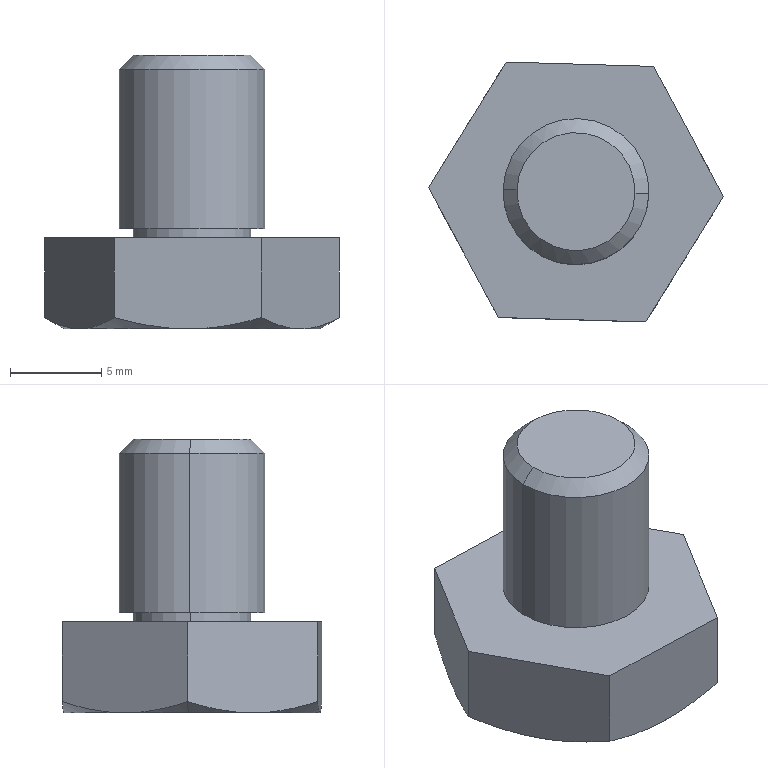Component | SolidWorks | STEHN14-1 | 1 solid | 23 faces | box 16.16 x 14.23 x 15 mm | volume 1333 mm3 | plane 10 | cone 9 | cylinder 4 | commonest cylinder face diameters 8 x2 6.466 x2 | material SUJ2
STEP:
#1=COLOUR_RGB('',0.7922,0.8196,0.9333);
#2=FILL_AREA_STYLE_COLOUR('',#1);
#3=FILL_AREA_STYLE('',(#2));
#4=SURFACE_STYLE_FILL_AREA(#3);
#5=SURFACE_SIDE_STYLE('',(#4));
#6=SURFACE_STYLE_USAGE(.BOTH.,#5);
#7=PRESENTATION_STYLE_ASSIGNMENT((#6));
#8=CARTESIAN_POINT('',(17.281,6.304,-9.769));
#9=VERTEX_POINT('',#8);
#10=CARTESIAN_POINT('',(17.322,6.441,-9.769));
#11=VERTEX_POINT('',#10);
#12=CARTESIAN_POINT('',(17.556,6.296,-9.769));
#13=DIRECTION('',(0.,-0.,-1.));
#14=DIRECTION('',(0.9996,-0.02982,0.));
#15=AXIS2_PLACEMENT_3D('',#12,#13,#14);
#16=CIRCLE('',#15,0.2756);
#17=EDGE_CURVE('',#9,#11,#16,.T.);
#18=ORIENTED_EDGE('',*,*,#17,.F.);
#19=CARTESIAN_POINT('',(17.238,6.305,-9.744));
#20=VERTEX_POINT('',#19);
#21=CARTESIAN_POINT('',(17.237,6.305,-9.744));
#22=DIRECTION('',(-0.8656,0.02582,0.5));
#23=VECTOR('',#22,39.37);
#24=LINE('',#21,#23);
#25=EDGE_CURVE('',#9,#20,#24,.T.);
#26=ORIENTED_EDGE('',*,*,#25,.T.);
#27=CARTESIAN_POINT('',(17.322,6.441,-9.769));
#28=CARTESIAN_POINT('',(17.315,6.429,-9.769));
#29=CARTESIAN_POINT('',(17.307,6.418,-9.768));
#30=CARTESIAN_POINT('',(17.293,6.395,-9.766));
#31=CARTESIAN_POINT('',(17.286,6.384,-9.764));
#32=CARTESIAN_POINT('',(17.265,6.35,-9.758));
#33=CARTESIAN_POINT('',(17.252,6.327,-9.752));
#34=CARTESIAN_POINT('',(17.238,6.305,-9.744));
#35=B_SPLINE_CURVE_WITH_KNOTS('',3,(#27,#28,#29,#30,#31,#32,#33,#34),.UNSPECIFIED.,.F.,.F.,(4,2,2,4),(0.00409,0.005108,0.006127,0.008164),.UNSPECIFIED.);
#36=EDGE_CURVE('',#11,#20,#35,.T.);
#37=ORIENTED_EDGE('',*,*,#36,.F.);
#38=EDGE_LOOP('',(#18,#26,#37));
#39=FACE_OUTER_BOUND('',#38,.T.);
#40=CARTESIAN_POINT('',(17.556,6.296,-9.744));
#41=DIRECTION('',(-0.,0.,1.));
#42=DIRECTION('',(-0.9996,0.02982,0.));
#43=AXIS2_PLACEMENT_3D('',#40,#41,#42);
#44=CONICAL_SURFACE('',#43,0.3189,1.047);
#45=ADVANCED_FACE('',(#39),#44,.T.);
#46=CARTESIAN_POINT('',(17.683,6.292,-9.178));
#47=VERTEX_POINT('',#46);
#48=CARTESIAN_POINT('',(17.429,6.3,-9.178));
#49=VERTEX_POINT('',#48);
#50=CARTESIAN_POINT('',(17.556,6.296,-9.178));
#51=DIRECTION('',(0.,-0.,-1.));
#52=DIRECTION('',(0.9996,-0.02982,0.));
#53=AXIS2_PLACEMENT_3D('',#50,#51,#52);
#54=CIRCLE('',#53,0.1273);
#55=EDGE_CURVE('',#47,#49,#54,.T.);
#56=ORIENTED_EDGE('',*,*,#55,.T.);
#57=CARTESIAN_POINT('',(17.399,6.301,-9.209));
#58=VERTEX_POINT('',#57);
#59=CARTESIAN_POINT('',(17.429,6.3,-9.178));
#60=DIRECTION('',(-0.7068,0.02108,-0.7071));
#61=VECTOR('',#60,39.37);
#62=LINE('',#59,#61);
#63=EDGE_CURVE('',#49,#58,#62,.T.);
#64=ORIENTED_EDGE('',*,*,#63,.T.);
#65=CARTESIAN_POINT('',(17.714,6.291,-9.209));
#66=VERTEX_POINT('',#65);
#67=CARTESIAN_POINT('',(17.556,6.296,-9.209));
#68=DIRECTION('',(0.,-0.,-1.));
#69=DIRECTION('',(0.9996,-0.02982,0.));
#70=AXIS2_PLACEMENT_3D('',#67,#68,#69);
#71=CIRCLE('',#70,0.1575);
#72=EDGE_CURVE('',#66,#58,#71,.T.);
#73=ORIENTED_EDGE('',*,*,#72,.F.);
#74=CARTESIAN_POINT('',(17.683,6.292,-9.178));
#75=DIRECTION('',(0.7068,-0.02108,-0.7071));
#76=VECTOR('',#75,39.37);
#77=LINE('',#74,#76);
#78=EDGE_CURVE('',#47,#66,#77,.T.);
#79=ORIENTED_EDGE('',*,*,#78,.F.);
#80=EDGE_LOOP('',(#56,#64,#73,#79));
#81=FACE_OUTER_BOUND('',#80,.T.);
#82=CARTESIAN_POINT('',(17.556,6.296,-9.178));
#83=DIRECTION('',(0.,-0.,-1.));
#84=DIRECTION('',(0.9996,-0.02982,0.));
#85=AXIS2_PLACEMENT_3D('',#82,#83,#84);
#86=CONICAL_SURFACE('',#85,0.1273,0.7854);
#87=ADVANCED_FACE('',(#81),#86,.T.);
#88=ORIENTED_EDGE('',*,*,#72,.T.);
#89=CARTESIAN_POINT('',(17.399,6.301,-9.552));
#90=VERTEX_POINT('',#89);
#91=CARTESIAN_POINT('',(17.399,6.301,-9.178));
#92=DIRECTION('',(0.,-0.,-1.));
#93=VECTOR('',#92,39.37);
#94=LINE('',#91,#93);
#95=EDGE_CURVE('',#58,#90,#94,.T.);
#96=ORIENTED_EDGE('',*,*,#95,.T.);
#97=CARTESIAN_POINT('',(17.714,6.291,-9.552));
#98=VERTEX_POINT('',#97);
#99=CARTESIAN_POINT('',(17.556,6.296,-9.552));
#100=DIRECTION('',(0.,-0.,-1.));
#101=DIRECTION('',(0.9996,-0.02982,0.));
#102=AXIS2_PLACEMENT_3D('',#99,#100,#101);
#103=CIRCLE('',#102,0.1575);
#104=EDGE_CURVE('',#98,#90,#103,.T.);
#105=ORIENTED_EDGE('',*,*,#104,.F.);
#106=CARTESIAN_POINT('',(17.714,6.291,-9.178));
#107=DIRECTION('',(0.,-0.,-1.));
#108=VECTOR('',#107,39.37);
#109=LINE('',#106,#108);
#110=EDGE_CURVE('',#66,#98,#109,.T.);
#111=ORIENTED_EDGE('',*,*,#110,.F.);
#112=EDGE_LOOP('',(#88,#96,#105,#111));
#113=FACE_OUTER_BOUND('',#112,.T.);
#114=CARTESIAN_POINT('',(17.556,6.296,-9.178));
#115=DIRECTION('',(0.,-0.,-1.));
#116=DIRECTION('',(0.9996,-0.02982,0.));
#117=AXIS2_PLACEMENT_3D('',#114,#115,#116);
#118=CYLINDRICAL_SURFACE('',#117,0.1575);
#119=ADVANCED_FACE('',(#113),#118,.T.);
#120=CARTESIAN_POINT('',(17.683,6.292,-9.552));
#121=VERTEX_POINT('',#120);
#122=CARTESIAN_POINT('',(17.429,6.3,-9.552));
#123=VERTEX_POINT('',#122);
#124=CARTESIAN_POINT('',(17.556,6.296,-9.552));
#125=DIRECTION('',(0.,-0.,-1.));
#126=DIRECTION('',(0.9996,-0.02982,0.));
#127=AXIS2_PLACEMENT_3D('',#124,#125,#126);
#128=CIRCLE('',#127,0.1273);
#129=EDGE_CURVE('',#121,#123,#128,.T.);
#130=ORIENTED_EDGE('',*,*,#129,.T.);
#131=CARTESIAN_POINT('',(17.429,6.3,-9.572));
#132=VERTEX_POINT('',#131);
#133=CARTESIAN_POINT('',(17.429,6.3,-9.178));
#134=DIRECTION('',(0.,-0.,-1.));
#135=VECTOR('',#134,39.37);
#136=LINE('',#133,#135);
#137=EDGE_CURVE('',#123,#132,#136,.T.);
#138=ORIENTED_EDGE('',*,*,#137,.T.);
#139=CARTESIAN_POINT('',(17.683,6.292,-9.572));
#140=VERTEX_POINT('',#139);
#141=CARTESIAN_POINT('',(17.556,6.296,-9.572));
#142=DIRECTION('',(0.,-0.,-1.));
#143=DIRECTION('',(0.9996,-0.02982,0.));
#144=AXIS2_PLACEMENT_3D('',#141,#142,#143);
#145=CIRCLE('',#144,0.1273);
#146=EDGE_CURVE('',#140,#132,#145,.T.);
#147=ORIENTED_EDGE('',*,*,#146,.F.);
#148=CARTESIAN_POINT('',(17.683,6.292,-9.178));
#149=DIRECTION('',(0.,-0.,-1.));
#150=VECTOR('',#149,39.37);
#151=LINE('',#148,#150);
#152=EDGE_CURVE('',#121,#140,#151,.T.);
#153=ORIENTED_EDGE('',*,*,#152,.F.);
#154=EDGE_LOOP('',(#130,#138,#147,#153));
#155=FACE_OUTER_BOUND('',#154,.T.);
#156=CARTESIAN_POINT('',(17.556,6.296,-9.178));
#157=DIRECTION('',(0.,-0.,-1.));
#158=DIRECTION('',(0.9996,-0.02982,0.));
#159=AXIS2_PLACEMENT_3D('',#156,#157,#158);
#160=CYLINDRICAL_SURFACE('',#159,0.1273);
#161=ADVANCED_FACE('',(#155),#160,.T.);
#162=ORIENTED_EDGE('',*,*,#146,.T.);
#163=CARTESIAN_POINT('',(17.556,6.296,-9.572));
#164=DIRECTION('',(0.,-0.,-1.));
#165=DIRECTION('',(0.9996,-0.02982,0.));
#166=AXIS2_PLACEMENT_3D('',#163,#164,#165);
#167=CIRCLE('',#166,0.1273);
#168=EDGE_CURVE('',#132,#140,#167,.T.);
#169=ORIENTED_EDGE('',*,*,#168,.T.);
#170=EDGE_LOOP('',(#162,#169));
#171=FACE_BOUND('',#170,.T.);
#172=CARTESIAN_POINT('',(17.238,6.305,-9.572));
#173=VERTEX_POINT('',#172);
#174=CARTESIAN_POINT('',(17.405,6.576,-9.572));
#175=VERTEX_POINT('',#174);
#176=CARTESIAN_POINT('',(17.238,6.305,-9.572));
#177=DIRECTION('',(0.5256,0.8507,0.));
#178=VECTOR('',#177,39.37);
#179=LINE('',#176,#178);
#180=EDGE_CURVE('',#173,#175,#179,.T.);
#181=ORIENTED_EDGE('',*,*,#180,.F.);
#182=CARTESIAN_POINT('',(17.389,6.025,-9.572));
#183=VERTEX_POINT('',#182);
#184=CARTESIAN_POINT('',(17.389,6.025,-9.572));
#185=DIRECTION('',(-0.474,0.8805,-0.));
#186=VECTOR('',#185,39.37);
#187=LINE('',#184,#186);
#188=EDGE_CURVE('',#183,#173,#187,.T.);
#189=ORIENTED_EDGE('',*,*,#188,.F.);
#190=CARTESIAN_POINT('',(17.707,6.016,-9.572));
#191=VERTEX_POINT('',#190);
#192=CARTESIAN_POINT('',(17.707,6.016,-9.572));
#193=DIRECTION('',(-0.9996,0.02982,-0.));
#194=VECTOR('',#193,39.37);
#195=LINE('',#192,#194);
#196=EDGE_CURVE('',#191,#183,#195,.T.);
#197=ORIENTED_EDGE('',*,*,#196,.F.);
#198=CARTESIAN_POINT('',(17.874,6.286,-9.572));
#199=VERTEX_POINT('',#198);
#200=CARTESIAN_POINT('',(17.874,6.286,-9.572));
#201=DIRECTION('',(-0.5256,-0.8507,-0.));
#202=VECTOR('',#201,39.37);
#203=LINE('',#200,#202);
#204=EDGE_CURVE('',#199,#191,#203,.T.);
#205=ORIENTED_EDGE('',*,*,#204,.F.);
#206=CARTESIAN_POINT('',(17.723,6.567,-9.572));
#207=VERTEX_POINT('',#206);
#208=CARTESIAN_POINT('',(17.723,6.567,-9.572));
#209=DIRECTION('',(0.474,-0.8805,0.));
#210=VECTOR('',#209,39.37);
#211=LINE('',#208,#210);
#212=EDGE_CURVE('',#207,#199,#211,.T.);
#213=ORIENTED_EDGE('',*,*,#212,.F.);
#214=CARTESIAN_POINT('',(17.405,6.576,-9.572));
#215=DIRECTION('',(0.9996,-0.02982,0.));
#216=VECTOR('',#215,39.37);
#217=LINE('',#214,#216);
#218=EDGE_CURVE('',#175,#207,#217,.T.);
#219=ORIENTED_EDGE('',*,*,#218,.F.);
#220=EDGE_LOOP('',(#181,#189,#197,#205,#213,#219));
#221=FACE_OUTER_BOUND('',#220,.T.);
#222=CARTESIAN_POINT('',(17.547,5.977,-9.572));
#223=DIRECTION('',(0.,-0.,-1.));
#224=DIRECTION('',(0.9996,-0.02982,0.));
#225=AXIS2_PLACEMENT_3D('',#222,#223,#224);
#226=PLANE('',#225);
#227=ADVANCED_FACE('',(#171,#221),#226,.F.);
#228=ORIENTED_EDGE('',*,*,#137,.F.);
#229=CARTESIAN_POINT('',(17.556,6.296,-9.552));
#230=DIRECTION('',(0.,-0.,-1.));
#231=DIRECTION('',(0.9996,-0.02982,0.));
#232=AXIS2_PLACEMENT_3D('',#229,#230,#231);
#233=CIRCLE('',#232,0.1273);
#234=EDGE_CURVE('',#123,#121,#233,.T.);
#235=ORIENTED_EDGE('',*,*,#234,.T.);
#236=ORIENTED_EDGE('',*,*,#152,.T.);
#237=ORIENTED_EDGE('',*,*,#168,.F.);
#238=EDGE_LOOP('',(#228,#235,#236,#237));
#239=FACE_OUTER_BOUND('',#238,.T.);
#240=CARTESIAN_POINT('',(17.556,6.296,-9.178));
#241=DIRECTION('',(0.,-0.,-1.));
#242=DIRECTION('',(0.9996,-0.02982,0.));
#243=AXIS2_PLACEMENT_3D('',#240,#241,#242);
#244=CYLINDRICAL_SURFACE('',#243,0.1273);
#245=ADVANCED_FACE('',(#239),#244,.T.);
#246=ORIENTED_EDGE('',*,*,#129,.F.);
#247=ORIENTED_EDGE('',*,*,#234,.F.);
#248=EDGE_LOOP('',(#246,#247));
#249=FACE_BOUND('',#248,.T.);
#250=ORIENTED_EDGE('',*,*,#104,.T.);
#251=CARTESIAN_POINT('',(17.556,6.296,-9.552));
#252=DIRECTION('',(0.,-0.,-1.));
#253=DIRECTION('',(0.9996,-0.02982,0.));
#254=AXIS2_PLACEMENT_3D('',#251,#252,#253);
#255=CIRCLE('',#254,0.1575);
#256=EDGE_CURVE('',#90,#98,#255,.T.);
#257=ORIENTED_EDGE('',*,*,#256,.T.);
#258=EDGE_LOOP('',(#250,#257));
#259=FACE_OUTER_BOUND('',#258,.T.);
#260=CARTESIAN_POINT('',(17.552,6.169,-9.552));
#261=DIRECTION('',(-0.,0.,1.));
#262=DIRECTION('',(-0.9996,0.02982,-0.));
#263=AXIS2_PLACEMENT_3D('',#260,#261,#262);
#264=PLANE('',#263);
#265=ADVANCED_FACE('',(#249,#259),#264,.F.);
#266=ORIENTED_EDGE('',*,*,#95,.F.);
#267=CARTESIAN_POINT('',(17.556,6.296,-9.209));
#268=DIRECTION('',(0.,-0.,-1.));
#269=DIRECTION('',(0.9996,-0.02982,0.));
#270=AXIS2_PLACEMENT_3D('',#267,#268,#269);
#271=CIRCLE('',#270,0.1575);
#272=EDGE_CURVE('',#58,#66,#271,.T.);
#273=ORIENTED_EDGE('',*,*,#272,.T.);
#274=ORIENTED_EDGE('',*,*,#110,.T.);
#275=ORIENTED_EDGE('',*,*,#256,.F.);
#276=EDGE_LOOP('',(#266,#273,#274,#275));
#277=FACE_OUTER_BOUND('',#276,.T.);
#278=CARTESIAN_POINT('',(17.556,6.296,-9.178));
#279=DIRECTION('',(0.,-0.,-1.));
#280=DIRECTION('',(0.9996,-0.02982,0.));
#281=AXIS2_PLACEMENT_3D('',#278,#279,#280);
#282=CYLINDRICAL_SURFACE('',#281,0.1575);
#283=ADVANCED_FACE('',(#277),#282,.T.);
#284=ORIENTED_EDGE('',*,*,#63,.F.);
#285=CARTESIAN_POINT('',(17.556,6.296,-9.178));
#286=DIRECTION('',(0.,-0.,-1.));
#287=DIRECTION('',(0.9996,-0.02982,0.));
#288=AXIS2_PLACEMENT_3D('',#285,#286,#287);
#289=CIRCLE('',#288,0.1273);
#290=EDGE_CURVE('',#49,#47,#289,.T.);
#291=ORIENTED_EDGE('',*,*,#290,.T.);
#292=ORIENTED_EDGE('',*,*,#78,.T.);
#293=ORIENTED_EDGE('',*,*,#272,.F.);
#294=EDGE_LOOP('',(#284,#291,#292,#293));
#295=FACE_OUTER_BOUND('',#294,.T.);
#296=CARTESIAN_POINT('',(17.556,6.296,-9.178));
#297=DIRECTION('',(0.,-0.,-1.));
#298=DIRECTION('',(0.9996,-0.02982,0.));
#299=AXIS2_PLACEMENT_3D('',#296,#297,#298);
#300=CONICAL_SURFACE('',#299,0.1273,0.7854);
#301=ADVANCED_FACE('',(#295),#300,.T.);
#302=ORIENTED_EDGE('',*,*,#55,.F.);
#303=ORIENTED_EDGE('',*,*,#290,.F.);
#304=EDGE_LOOP('',(#302,#303));
#305=FACE_OUTER_BOUND('',#304,.T.);
#306=CARTESIAN_POINT('',(17.552,6.169,-9.178));
#307=DIRECTION('',(0.,-0.,-1.));
#308=DIRECTION('',(0.9996,-0.02982,0.));
#309=AXIS2_PLACEMENT_3D('',#306,#307,#308);
#310=PLANE('',#309);
#311=ADVANCED_FACE('',(#305),#310,.F.);
#312=CARTESIAN_POINT('',(17.405,6.576,-9.744));
#313=VERTEX_POINT('',#312);
#314=CARTESIAN_POINT('',(17.405,6.576,-9.744));
#315=CARTESIAN_POINT('',(17.392,6.554,-9.752));
#316=CARTESIAN_POINT('',(17.378,6.532,-9.758));
#317=CARTESIAN_POINT('',(17.35,6.487,-9.767));
#318=CARTESIAN_POINT('',(17.336,6.464,-9.769));
#319=CARTESIAN_POINT('',(17.322,6.441,-9.769));
#320=B_SPLINE_CURVE_WITH_KNOTS('',3,(#314,#315,#316,#317,#318,#319),.UNSPECIFIED.,.F.,.F.,(4,2,4),(0.00000024,0.002045,0.00409),.UNSPECIFIED.);
#321=EDGE_CURVE('',#313,#11,#320,.T.);
#322=ORIENTED_EDGE('',*,*,#321,.T.);
#323=ORIENTED_EDGE('',*,*,#36,.T.);
#324=CARTESIAN_POINT('',(17.238,6.305,-9.572));
#325=DIRECTION('',(0.,-0.,-1.));
#326=VECTOR('',#325,39.37);
#327=LINE('',#324,#326);
#328=EDGE_CURVE('',#173,#20,#327,.T.);
#329=ORIENTED_EDGE('',*,*,#328,.F.);
#330=ORIENTED_EDGE('',*,*,#180,.T.);
#331=CARTESIAN_POINT('',(17.405,6.576,-9.572));
#332=DIRECTION('',(0.,-0.,-1.));
#333=VECTOR('',#332,39.37);
#334=LINE('',#331,#333);
#335=EDGE_CURVE('',#175,#313,#334,.T.);
#336=ORIENTED_EDGE('',*,*,#335,.T.);
#337=EDGE_LOOP('',(#322,#323,#329,#330,#336));
#338=FACE_OUTER_BOUND('',#337,.T.);
#339=CARTESIAN_POINT('',(17.238,6.305,-9.572));
#340=DIRECTION('',(-0.8507,0.5256,-0.));
#341=DIRECTION('',(-0.5256,-0.8507,-0.));
#342=AXIS2_PLACEMENT_3D('',#339,#340,#341);
#343=PLANE('',#342);
#344=ADVANCED_FACE('',(#338),#343,.T.);
#345=CARTESIAN_POINT('',(17.313,6.165,-9.769));
#346=VERTEX_POINT('',#345);
#347=CARTESIAN_POINT('',(17.238,6.305,-9.744));
#348=CARTESIAN_POINT('',(17.25,6.282,-9.752));
#349=CARTESIAN_POINT('',(17.263,6.259,-9.758));
#350=CARTESIAN_POINT('',(17.288,6.213,-9.767));
#351=CARTESIAN_POINT('',(17.301,6.189,-9.769));
#352=CARTESIAN_POINT('',(17.313,6.165,-9.769));
#353=B_SPLINE_CURVE_WITH_KNOTS('',3,(#347,#348,#349,#350,#351,#352),.UNSPECIFIED.,.F.,.F.,(4,2,4),(0.00000024,0.002045,0.00409),.UNSPECIFIED.);
#354=EDGE_CURVE('',#20,#346,#353,.T.);
#355=ORIENTED_EDGE('',*,*,#354,.T.);
#356=CARTESIAN_POINT('',(17.389,6.025,-9.744));
#357=VERTEX_POINT('',#356);
#358=CARTESIAN_POINT('',(17.313,6.165,-9.769));
#359=CARTESIAN_POINT('',(17.32,6.153,-9.769));
#360=CARTESIAN_POINT('',(17.326,6.141,-9.768));
#361=CARTESIAN_POINT('',(17.339,6.118,-9.766));
#362=CARTESIAN_POINT('',(17.345,6.106,-9.764));
#363=CARTESIAN_POINT('',(17.364,6.071,-9.758));
#364=CARTESIAN_POINT('',(17.377,6.048,-9.752));
#365=CARTESIAN_POINT('',(17.389,6.025,-9.744));
#366=B_SPLINE_CURVE_WITH_KNOTS('',3,(#358,#359,#360,#361,#362,#363,#364,#365),.UNSPECIFIED.,.F.,.F.,(4,2,2,4),(0.00409,0.005108,0.006127,0.008164),.UNSPECIFIED.);
#367=EDGE_CURVE('',#346,#357,#366,.T.);
#368=ORIENTED_EDGE('',*,*,#367,.T.);
#369=CARTESIAN_POINT('',(17.389,6.025,-9.572));
#370=DIRECTION('',(0.,-0.,-1.));
#371=VECTOR('',#370,39.37);
#372=LINE('',#369,#371);
#373=EDGE_CURVE('',#183,#357,#372,.T.);
#374=ORIENTED_EDGE('',*,*,#373,.F.);
#375=ORIENTED_EDGE('',*,*,#188,.T.);
#376=ORIENTED_EDGE('',*,*,#328,.T.);
#377=EDGE_LOOP('',(#355,#368,#374,#375,#376));
#378=FACE_OUTER_BOUND('',#377,.T.);
#379=CARTESIAN_POINT('',(17.389,6.025,-9.572));
#380=DIRECTION('',(-0.8805,-0.474,-0.));
#381=DIRECTION('',(0.474,-0.8805,0.));
#382=AXIS2_PLACEMENT_3D('',#379,#380,#381);
#383=PLANE('',#382);
#384=ADVANCED_FACE('',(#378),#383,.T.);
#385=CARTESIAN_POINT('',(17.548,6.02,-9.769));
#386=VERTEX_POINT('',#385);
#387=CARTESIAN_POINT('',(17.389,6.025,-9.744));
#388=CARTESIAN_POINT('',(17.415,6.024,-9.752));
#389=CARTESIAN_POINT('',(17.441,6.024,-9.758));
#390=CARTESIAN_POINT('',(17.494,6.022,-9.767));
#391=CARTESIAN_POINT('',(17.521,6.021,-9.769));
#392=CARTESIAN_POINT('',(17.548,6.02,-9.769));
#393=B_SPLINE_CURVE_WITH_KNOTS('',3,(#387,#388,#389,#390,#391,#392),.UNSPECIFIED.,.F.,.F.,(4,2,4),(0.007212,0.009256,0.0113),.UNSPECIFIED.);
#394=EDGE_CURVE('',#357,#386,#393,.T.);
#395=ORIENTED_EDGE('',*,*,#394,.T.);
#396=CARTESIAN_POINT('',(17.707,6.016,-9.744));
#397=VERTEX_POINT('',#396);
#398=CARTESIAN_POINT('',(17.548,6.02,-9.769));
#399=CARTESIAN_POINT('',(17.575,6.02,-9.769));
#400=CARTESIAN_POINT('',(17.602,6.019,-9.767));
#401=CARTESIAN_POINT('',(17.655,6.017,-9.758));
#402=CARTESIAN_POINT('',(17.681,6.016,-9.752));
#403=CARTESIAN_POINT('',(17.707,6.016,-9.744));
#404=B_SPLINE_CURVE_WITH_KNOTS('',3,(#398,#399,#400,#401,#402,#403),.UNSPECIFIED.,.F.,.F.,(4,2,4),(0.0113,0.01335,0.01539),.UNSPECIFIED.);
#405=EDGE_CURVE('',#386,#397,#404,.T.);
#406=ORIENTED_EDGE('',*,*,#405,.T.);
#407=CARTESIAN_POINT('',(17.707,6.016,-9.572));
#408=DIRECTION('',(0.,-0.,-1.));
#409=VECTOR('',#408,39.37);
#410=LINE('',#407,#409);
#411=EDGE_CURVE('',#191,#397,#410,.T.);
#412=ORIENTED_EDGE('',*,*,#411,.F.);
#413=ORIENTED_EDGE('',*,*,#196,.T.);
#414=ORIENTED_EDGE('',*,*,#373,.T.);
#415=EDGE_LOOP('',(#395,#406,#412,#413,#414));
#416=FACE_OUTER_BOUND('',#415,.T.);
#417=CARTESIAN_POINT('',(17.707,6.016,-9.572));
#418=DIRECTION('',(-0.02982,-0.9996,-0.));
#419=DIRECTION('',(0.9996,-0.02982,0.));
#420=AXIS2_PLACEMENT_3D('',#417,#418,#419);
#421=PLANE('',#420);
#422=ADVANCED_FACE('',(#416),#421,.T.);
#423=CARTESIAN_POINT('',(17.791,6.151,-9.769));
#424=VERTEX_POINT('',#423);
#425=CARTESIAN_POINT('',(17.707,6.016,-9.744));
#426=CARTESIAN_POINT('',(17.721,6.038,-9.752));
#427=CARTESIAN_POINT('',(17.734,6.06,-9.758));
#428=CARTESIAN_POINT('',(17.762,6.105,-9.767));
#429=CARTESIAN_POINT('',(17.776,6.128,-9.769));
#430=CARTESIAN_POINT('',(17.791,6.151,-9.769));
#431=B_SPLINE_CURVE_WITH_KNOTS('',3,(#425,#426,#427,#428,#429,#430),.UNSPECIFIED.,.F.,.F.,(4,2,4),(0.00000024,0.002045,0.00409),.UNSPECIFIED.);
#432=EDGE_CURVE('',#397,#424,#431,.T.);
#433=ORIENTED_EDGE('',*,*,#432,.T.);
#434=CARTESIAN_POINT('',(17.874,6.286,-9.744));
#435=VERTEX_POINT('',#434);
#436=CARTESIAN_POINT('',(17.791,6.151,-9.769));
#437=CARTESIAN_POINT('',(17.798,6.163,-9.769));
#438=CARTESIAN_POINT('',(17.805,6.174,-9.768));
#439=CARTESIAN_POINT('',(17.819,6.197,-9.766));
#440=CARTESIAN_POINT('',(17.826,6.208,-9.764));
#441=CARTESIAN_POINT('',(17.847,6.242,-9.758));
#442=CARTESIAN_POINT('',(17.861,6.264,-9.752));
#443=CARTESIAN_POINT('',(17.874,6.286,-9.744));
#444=B_SPLINE_CURVE_WITH_KNOTS('',3,(#436,#437,#438,#439,#440,#441,#442,#443),.UNSPECIFIED.,.F.,.F.,(4,2,2,4),(0.00409,0.005108,0.006127,0.008164),.UNSPECIFIED.);
#445=EDGE_CURVE('',#424,#435,#444,.T.);
#446=ORIENTED_EDGE('',*,*,#445,.T.);
#447=CARTESIAN_POINT('',(17.874,6.286,-9.572));
#448=DIRECTION('',(0.,-0.,-1.));
#449=VECTOR('',#448,39.37);
#450=LINE('',#447,#449);
#451=EDGE_CURVE('',#199,#435,#450,.T.);
#452=ORIENTED_EDGE('',*,*,#451,.F.);
#453=ORIENTED_EDGE('',*,*,#204,.T.);
#454=ORIENTED_EDGE('',*,*,#411,.T.);
#455=EDGE_LOOP('',(#433,#446,#452,#453,#454));
#456=FACE_OUTER_BOUND('',#455,.T.);
#457=CARTESIAN_POINT('',(17.874,6.286,-9.572));
#458=DIRECTION('',(0.8507,-0.5256,0.));
#459=DIRECTION('',(0.5256,0.8507,0.));
#460=AXIS2_PLACEMENT_3D('',#457,#458,#459);
#461=PLANE('',#460);
#462=ADVANCED_FACE('',(#456),#461,.T.);
#463=CARTESIAN_POINT('',(17.799,6.427,-9.769));
#464=VERTEX_POINT('',#463);
#465=CARTESIAN_POINT('',(17.874,6.286,-9.744));
#466=CARTESIAN_POINT('',(17.862,6.309,-9.752));
#467=CARTESIAN_POINT('',(17.849,6.332,-9.758));
#468=CARTESIAN_POINT('',(17.824,6.379,-9.767));
#469=CARTESIAN_POINT('',(17.812,6.403,-9.769));
#470=CARTESIAN_POINT('',(17.799,6.427,-9.769));
#471=B_SPLINE_CURVE_WITH_KNOTS('',3,(#465,#466,#467,#468,#469,#470),.UNSPECIFIED.,.F.,.F.,(4,2,4),(0.00000024,0.002045,0.00409),.UNSPECIFIED.);
#472=EDGE_CURVE('',#435,#464,#471,.T.);
#473=ORIENTED_EDGE('',*,*,#472,.T.);
#474=CARTESIAN_POINT('',(17.723,6.567,-9.744));
#475=VERTEX_POINT('',#474);
#476=CARTESIAN_POINT('',(17.799,6.427,-9.769));
#477=CARTESIAN_POINT('',(17.792,6.438,-9.769));
#478=CARTESIAN_POINT('',(17.786,6.45,-9.768));
#479=CARTESIAN_POINT('',(17.773,6.474,-9.766));
#480=CARTESIAN_POINT('',(17.767,6.486,-9.764));
#481=CARTESIAN_POINT('',(17.748,6.521,-9.758));
#482=CARTESIAN_POINT('',(17.736,6.544,-9.752));
#483=CARTESIAN_POINT('',(17.723,6.567,-9.744));
#484=B_SPLINE_CURVE_WITH_KNOTS('',3,(#476,#477,#478,#479,#480,#481,#482,#483),.UNSPECIFIED.,.F.,.F.,(4,2,2,4),(0.00409,0.005108,0.006127,0.008164),.UNSPECIFIED.);
#485=EDGE_CURVE('',#464,#475,#484,.T.);
#486=ORIENTED_EDGE('',*,*,#485,.T.);
#487=CARTESIAN_POINT('',(17.723,6.567,-9.572));
#488=DIRECTION('',(0.,-0.,-1.));
#489=VECTOR('',#488,39.37);
#490=LINE('',#487,#489);
#491=EDGE_CURVE('',#207,#475,#490,.T.);
#492=ORIENTED_EDGE('',*,*,#491,.F.);
#493=ORIENTED_EDGE('',*,*,#212,.T.);
#494=ORIENTED_EDGE('',*,*,#451,.T.);
#495=EDGE_LOOP('',(#473,#486,#492,#493,#494));
#496=FACE_OUTER_BOUND('',#495,.T.);
#497=CARTESIAN_POINT('',(17.723,6.567,-9.572));
#498=DIRECTION('',(0.8805,0.474,0.));
#499=DIRECTION('',(-0.474,0.8805,-0.));
#500=AXIS2_PLACEMENT_3D('',#497,#498,#499);
#501=PLANE('',#500);
#502=ADVANCED_FACE('',(#496),#501,.T.);
#503=CARTESIAN_POINT('',(17.564,6.571,-9.769));
#504=VERTEX_POINT('',#503);
#505=CARTESIAN_POINT('',(17.723,6.567,-9.744));
#506=CARTESIAN_POINT('',(17.698,6.567,-9.752));
#507=CARTESIAN_POINT('',(17.672,6.568,-9.758));
#508=CARTESIAN_POINT('',(17.618,6.57,-9.767));
#509=CARTESIAN_POINT('',(17.591,6.571,-9.769));
#510=CARTESIAN_POINT('',(17.564,6.571,-9.769));
#511=B_SPLINE_CURVE_WITH_KNOTS('',3,(#505,#506,#507,#508,#509,#510),.UNSPECIFIED.,.F.,.F.,(4,2,4),(0.002961,0.005001,0.007041),.UNSPECIFIED.);
#512=EDGE_CURVE('',#475,#504,#511,.T.);
#513=ORIENTED_EDGE('',*,*,#512,.T.);
#514=CARTESIAN_POINT('',(17.564,6.571,-9.769));
#515=CARTESIAN_POINT('',(17.537,6.572,-9.769));
#516=CARTESIAN_POINT('',(17.511,6.573,-9.767));
#517=CARTESIAN_POINT('',(17.458,6.575,-9.758));
#518=CARTESIAN_POINT('',(17.431,6.575,-9.752));
#519=CARTESIAN_POINT('',(17.405,6.576,-9.744));
#520=B_SPLINE_CURVE_WITH_KNOTS('',3,(#514,#515,#516,#517,#518,#519),.UNSPECIFIED.,.F.,.F.,(4,2,4),(0.007041,0.00908,0.01112),.UNSPECIFIED.);
#521=EDGE_CURVE('',#504,#313,#520,.T.);
#522=ORIENTED_EDGE('',*,*,#521,.T.);
#523=ORIENTED_EDGE('',*,*,#335,.F.);
#524=ORIENTED_EDGE('',*,*,#218,.T.);
#525=ORIENTED_EDGE('',*,*,#491,.T.);
#526=EDGE_LOOP('',(#513,#522,#523,#524,#525));
#527=FACE_OUTER_BOUND('',#526,.T.);
#528=CARTESIAN_POINT('',(17.405,6.576,-9.572));
#529=DIRECTION('',(0.02982,0.9996,0.));
#530=DIRECTION('',(-0.9996,0.02982,-0.));
#531=AXIS2_PLACEMENT_3D('',#528,#529,#530);
#532=PLANE('',#531);
#533=ADVANCED_FACE('',(#527),#532,.T.);
#534=ORIENTED_EDGE('',*,*,#445,.F.);
#535=CARTESIAN_POINT('',(17.556,6.296,-9.769));
#536=DIRECTION('',(0.,-0.,-1.));
#537=DIRECTION('',(0.9996,-0.02982,0.));
#538=AXIS2_PLACEMENT_3D('',#535,#536,#537);
#539=CIRCLE('',#538,0.2756);
#540=EDGE_CURVE('',#464,#424,#539,.T.);
#541=ORIENTED_EDGE('',*,*,#540,.F.);
#542=ORIENTED_EDGE('',*,*,#472,.F.);
#543=EDGE_LOOP('',(#534,#541,#542));
#544=FACE_OUTER_BOUND('',#543,.T.);
#545=CARTESIAN_POINT('',(17.556,6.296,-9.744));
#546=DIRECTION('',(-0.,0.,1.));
#547=DIRECTION('',(-0.9996,0.02982,0.));
#548=AXIS2_PLACEMENT_3D('',#545,#546,#547);
#549=CONICAL_SURFACE('',#548,0.3189,1.047);
#550=ADVANCED_FACE('',(#544),#549,.T.);
#551=ORIENTED_EDGE('',*,*,#485,.F.);
#552=CARTESIAN_POINT('',(17.556,6.296,-9.769));
#553=DIRECTION('',(0.,-0.,-1.));
#554=DIRECTION('',(0.9996,-0.02982,0.));
#555=AXIS2_PLACEMENT_3D('',#552,#553,#554);
#556=CIRCLE('',#555,0.2756);
#557=EDGE_CURVE('',#504,#464,#556,.T.);
#558=ORIENTED_EDGE('',*,*,#557,.F.);
#559=ORIENTED_EDGE('',*,*,#512,.F.);
#560=EDGE_LOOP('',(#551,#558,#559));
#561=FACE_OUTER_BOUND('',#560,.T.);
#562=CARTESIAN_POINT('',(17.556,6.296,-9.744));
#563=DIRECTION('',(-0.,0.,1.));
#564=DIRECTION('',(-0.9996,0.02982,0.));
#565=AXIS2_PLACEMENT_3D('',#562,#563,#564);
#566=CONICAL_SURFACE('',#565,0.3189,1.047);
#567=ADVANCED_FACE('',(#561),#566,.T.);
#568=ORIENTED_EDGE('',*,*,#25,.F.);
#569=CARTESIAN_POINT('',(17.556,6.296,-9.769));
#570=DIRECTION('',(0.,-0.,-1.));
#571=DIRECTION('',(0.9996,-0.02982,0.));
#572=AXIS2_PLACEMENT_3D('',#569,#570,#571);
#573=CIRCLE('',#572,0.2756);
#574=EDGE_CURVE('',#346,#9,#573,.T.);
#575=ORIENTED_EDGE('',*,*,#574,.F.);
#576=ORIENTED_EDGE('',*,*,#354,.F.);
#577=EDGE_LOOP('',(#568,#575,#576));
#578=FACE_OUTER_BOUND('',#577,.T.);
#579=CARTESIAN_POINT('',(17.556,6.296,-9.744));
#580=DIRECTION('',(-0.,0.,1.));
#581=DIRECTION('',(-0.9996,0.02982,0.));
#582=AXIS2_PLACEMENT_3D('',#579,#580,#581);
#583=CONICAL_SURFACE('',#582,0.3189,1.047);
#584=ADVANCED_FACE('',(#578),#583,.T.);
#585=ORIENTED_EDGE('',*,*,#367,.F.);
#586=CARTESIAN_POINT('',(17.556,6.296,-9.769));
#587=DIRECTION('',(0.,-0.,-1.));
#588=DIRECTION('',(0.9996,-0.02982,0.));
#589=AXIS2_PLACEMENT_3D('',#586,#587,#588);
#590=CIRCLE('',#589,0.2756);
#591=EDGE_CURVE('',#386,#346,#590,.T.);
#592=ORIENTED_EDGE('',*,*,#591,.F.);
#593=ORIENTED_EDGE('',*,*,#394,.F.);
#594=EDGE_LOOP('',(#585,#592,#593));
#595=FACE_OUTER_BOUND('',#594,.T.);
#596=CARTESIAN_POINT('',(17.556,6.296,-9.744));
#597=DIRECTION('',(-0.,0.,1.));
#598=DIRECTION('',(-0.9996,0.02982,0.));
#599=AXIS2_PLACEMENT_3D('',#596,#597,#598);
#600=CONICAL_SURFACE('',#599,0.3189,1.047);
#601=ADVANCED_FACE('',(#595),#600,.T.);
#602=ORIENTED_EDGE('',*,*,#405,.F.);
#603=CARTESIAN_POINT('',(17.556,6.296,-9.769));
#604=DIRECTION('',(0.,-0.,-1.));
#605=DIRECTION('',(0.9996,-0.02982,0.));
#606=AXIS2_PLACEMENT_3D('',#603,#604,#605);
#607=CIRCLE('',#606,0.2756);
#608=EDGE_CURVE('',#424,#386,#607,.T.);
#609=ORIENTED_EDGE('',*,*,#608,.F.);
#610=ORIENTED_EDGE('',*,*,#432,.F.);
#611=EDGE_LOOP('',(#602,#609,#610));
#612=FACE_OUTER_BOUND('',#611,.T.);
#613=CARTESIAN_POINT('',(17.556,6.296,-9.744));
#614=DIRECTION('',(-0.,0.,1.));
#615=DIRECTION('',(-0.9996,0.02982,0.));
#616=AXIS2_PLACEMENT_3D('',#613,#614,#615);
#617=CONICAL_SURFACE('',#616,0.3189,1.047);
#618=ADVANCED_FACE('',(#612),#617,.T.);
#619=ORIENTED_EDGE('',*,*,#608,.T.);
#620=ORIENTED_EDGE('',*,*,#591,.T.);
#621=ORIENTED_EDGE('',*,*,#574,.T.);
#622=ORIENTED_EDGE('',*,*,#17,.T.);
#623=CARTESIAN_POINT('',(17.556,6.296,-9.769));
#624=DIRECTION('',(0.,-0.,-1.));
#625=DIRECTION('',(0.9996,-0.02982,0.));
#626=AXIS2_PLACEMENT_3D('',#623,#624,#625);
#627=CIRCLE('',#626,0.2756);
#628=EDGE_CURVE('',#11,#504,#627,.T.);
#629=ORIENTED_EDGE('',*,*,#628,.T.);
#630=ORIENTED_EDGE('',*,*,#557,.T.);
#631=ORIENTED_EDGE('',*,*,#540,.T.);
#632=EDGE_LOOP('',(#619,#620,#621,#622,#629,#630,#631));
#633=FACE_OUTER_BOUND('',#632,.T.);
#634=CARTESIAN_POINT('',(17.556,6.296,-9.769));
#635=DIRECTION('',(-0.,0.,1.));
#636=DIRECTION('',(-0.9996,0.02982,-0.));
#637=AXIS2_PLACEMENT_3D('',#634,#635,#636);
#638=PLANE('',#637);
#639=ADVANCED_FACE('',(#633),#638,.F.);
#640=ORIENTED_EDGE('',*,*,#321,.F.);
#641=ORIENTED_EDGE('',*,*,#521,.F.);
#642=ORIENTED_EDGE('',*,*,#628,.F.);
#643=EDGE_LOOP('',(#640,#641,#642));
#644=FACE_OUTER_BOUND('',#643,.T.);
#645=CARTESIAN_POINT('',(17.556,6.296,-9.744));
#646=DIRECTION('',(-0.,0.,1.));
#647=DIRECTION('',(-0.9996,0.02982,0.));
#648=AXIS2_PLACEMENT_3D('',#645,#646,#647);
#649=CONICAL_SURFACE('',#648,0.3189,1.047);
#650=ADVANCED_FACE('',(#644),#649,.T.);
#651=CLOSED_SHELL('',(#45,#87,#119,#161,#227,#245,#265,#283,#301,#311,#344,#384,#422,#462,#502,#533,#550,#567,#584,#601,#618,#639,#650));
#652=MANIFOLD_SOLID_BREP('',#651);
#653=STYLED_ITEM('',(#7),#652);
#654=PRESENTATION_LAYER_ASSIGNMENT('','',(#653));
#655=CARTESIAN_POINT('',(0.,0.,0.));
#656=DIRECTION('',(0.,0.,1.));
#657=DIRECTION('',(1.,0.,0.));
#658=AXIS2_PLACEMENT_3D('',#655,#656,#657);
#659=(LENGTH_UNIT()NAMED_UNIT(*)SI_UNIT($,.METRE.));
#660=LENGTH_MEASURE_WITH_UNIT(LENGTH_MEASURE(0.0254),#659);
#661=DIMENSIONAL_EXPONENTS(1.,0.,0.,0.,0.,0.,0.);
#662=(CONVERSION_BASED_UNIT('',#660)LENGTH_UNIT()NAMED_UNIT(#661));
#663=UNCERTAINTY_MEASURE_WITH_UNIT(LENGTH_MEASURE(0.00001),#662,'','');
#664=(NAMED_UNIT(*)PLANE_ANGLE_UNIT()SI_UNIT($,.RADIAN.));
#665=(NAMED_UNIT(*)SI_UNIT($,.STERADIAN.)SOLID_ANGLE_UNIT());
#666=(GEOMETRIC_REPRESENTATION_CONTEXT(3)GLOBAL_UNCERTAINTY_ASSIGNED_CONTEXT((#663))GLOBAL_UNIT_ASSIGNED_CONTEXT((#662,#664,#665))REPRESENTATION_CONTEXT('',''));
#667=ADVANCED_BREP_SHAPE_REPRESENTATION('',(#652,#658),#666);
#668=(LENGTH_UNIT()NAMED_UNIT(*)SI_UNIT($,.METRE.));
#669=LENGTH_MEASURE_WITH_UNIT(LENGTH_MEASURE(0.0254),#668);
#670=DIMENSIONAL_EXPONENTS(1.,0.,0.,0.,0.,0.,0.);
#671=(CONVERSION_BASED_UNIT('',#669)LENGTH_UNIT()NAMED_UNIT(#670));
#672=UNCERTAINTY_MEASURE_WITH_UNIT(LENGTH_MEASURE(0.00001),#671,'','');
#673=(NAMED_UNIT(*)PLANE_ANGLE_UNIT()SI_UNIT($,.RADIAN.));
#674=(NAMED_UNIT(*)SI_UNIT($,.STERADIAN.)SOLID_ANGLE_UNIT());
#675=(GEOMETRIC_REPRESENTATION_CONTEXT(3)GLOBAL_UNCERTAINTY_ASSIGNED_CONTEXT((#672))GLOBAL_UNIT_ASSIGNED_CONTEXT((#671,#673,#674))REPRESENTATION_CONTEXT('',''));
#676=MECHANICAL_DESIGN_GEOMETRIC_PRESENTATION_REPRESENTATION('',(#653),#675);